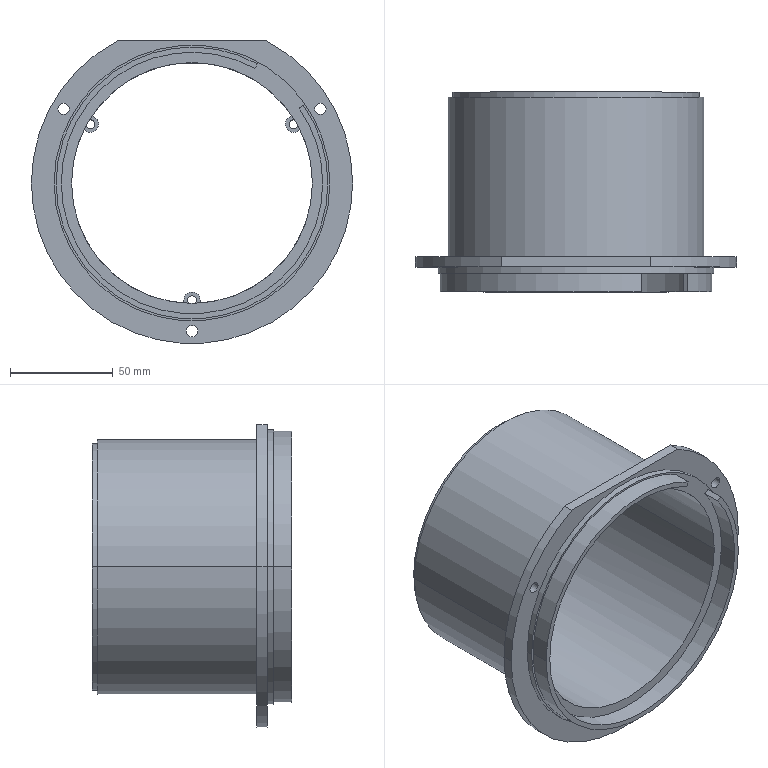Component | SolidWorks | Stator-1 | 1 solid | 54 faces | box 156 x 97 x 147 mm | volume 162812 mm3 | cylinder 33 | plane 21 | commonest cylinder face diameters 4.4 x6 5.5 x6 8 x4 127 x3 132 x3 156 x3 120 x2 134 x2